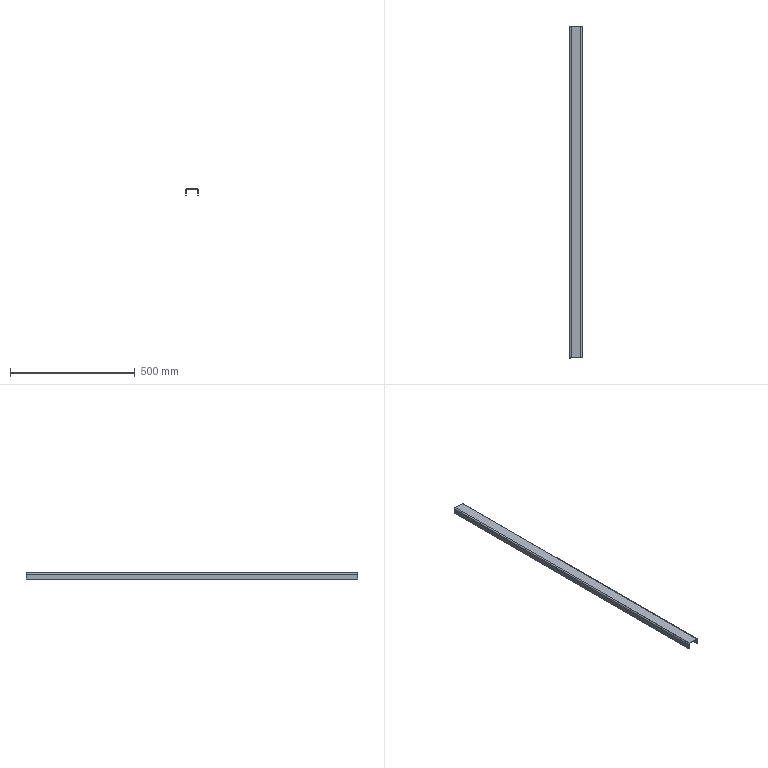Component | SolidWorks | BoxWelding-1_SupportChannelPlate-1 | 1 solid | 14 faces | box 50 x 1331 x 25 mm | volume 246412 mm3 | plane 10 | cylinder 4 | commonest cylinder face diameters 10 x2 6 x2
build123d program:
from build123d import *

# Parameters (mm, degrees)
EXTRUDE_THIN1_DEPTH = 665.5


with BuildPart() as part:
    # Sketch1 → Extrude-Thin1 (new, symmetric)
    with BuildSketch(Plane.XY):
        with BuildLine():
            Line((-25, 24), (-25, 4))
            ThreePointArc((-25, 4), (-23.536, 0.4645), (-20, -1))
            Line((-20, -1), (20, -1))
            ThreePointArc((20, -1), (23.536, 0.4645), (25, 4))
            Line((25, 4), (25, 24))
            Line((25, 24), (23, 24))
            Line((23, 24), (23, 4))
            ThreePointArc((23, 4), (22.121, 1.879), (20, 1))
            Line((20, 1), (-20, 1))
            ThreePointArc((-20, 1), (-22.121, 1.879), (-23, 4))
            Line((-23, 4), (-23, 24))
            Line((-23, 24), (-25, 24))
        make_face()
    extrude(amount=EXTRUDE_THIN1_DEPTH, both=True)


solid = part.part

# Placed as in the assembly
solid = solid.moved(Location((-103.378, 621.001, -155.987), (-90, 0, 0)))
STEP:
#1=COLOUR_RGB('',0.7922,0.8196,0.9333);
#2=FILL_AREA_STYLE_COLOUR('',#1);
#3=FILL_AREA_STYLE('',(#2));
#4=SURFACE_STYLE_FILL_AREA(#3);
#5=SURFACE_SIDE_STYLE('',(#4));
#6=SURFACE_STYLE_USAGE(.BOTH.,#5);
#7=PRESENTATION_STYLE_ASSIGNMENT((#6));
#8=CARTESIAN_POINT('',(-3.165,50.65,-6.299));
#9=VERTEX_POINT('',#8);
#10=CARTESIAN_POINT('',(-3.165,50.65,-7.086));
#11=VERTEX_POINT('',#10);
#12=CARTESIAN_POINT('',(-3.165,50.65,-7.086));
#13=DIRECTION('',(0.,-0.,-1.));
#14=VECTOR('',#13,39.37);
#15=LINE('',#12,#14);
#16=EDGE_CURVE('',#9,#11,#15,.T.);
#17=ORIENTED_EDGE('',*,*,#16,.T.);
#18=CARTESIAN_POINT('',(-3.165,-1.752,-7.086));
#19=VERTEX_POINT('',#18);
#20=CARTESIAN_POINT('',(-3.165,-1.752,-7.086));
#21=DIRECTION('',(-0.,1.,-0.));
#22=VECTOR('',#21,39.37);
#23=LINE('',#20,#22);
#24=EDGE_CURVE('',#19,#11,#23,.T.);
#25=ORIENTED_EDGE('',*,*,#24,.F.);
#26=CARTESIAN_POINT('',(-3.165,-1.752,-6.299));
#27=VERTEX_POINT('',#26);
#28=CARTESIAN_POINT('',(-3.165,-1.752,-7.086));
#29=DIRECTION('',(0.,-0.,-1.));
#30=VECTOR('',#29,39.37);
#31=LINE('',#28,#30);
#32=EDGE_CURVE('',#27,#19,#31,.T.);
#33=ORIENTED_EDGE('',*,*,#32,.F.);
#34=CARTESIAN_POINT('',(-3.165,-1.752,-6.299));
#35=DIRECTION('',(-0.,1.,-0.));
#36=VECTOR('',#35,39.37);
#37=LINE('',#34,#36);
#38=EDGE_CURVE('',#27,#9,#37,.T.);
#39=ORIENTED_EDGE('',*,*,#38,.T.);
#40=EDGE_LOOP('',(#17,#25,#33,#39));
#41=FACE_OUTER_BOUND('',#40,.T.);
#42=CARTESIAN_POINT('',(-3.165,-1.752,-7.086));
#43=DIRECTION('',(1.,0.,0.));
#44=DIRECTION('',(0.,-1.,0.));
#45=AXIS2_PLACEMENT_3D('',#42,#43,#44);
#46=PLANE('',#45);
#47=ADVANCED_FACE('',(#41),#46,.F.);
#48=CARTESIAN_POINT('',(-3.086,50.65,-7.086));
#49=VERTEX_POINT('',#48);
#50=CARTESIAN_POINT('',(-3.086,50.65,-7.086));
#51=DIRECTION('',(-1.,-0.,-0.));
#52=VECTOR('',#51,39.37);
#53=LINE('',#50,#52);
#54=EDGE_CURVE('',#49,#11,#53,.T.);
#55=ORIENTED_EDGE('',*,*,#54,.F.);
#56=CARTESIAN_POINT('',(-3.086,-1.752,-7.086));
#57=VERTEX_POINT('',#56);
#58=CARTESIAN_POINT('',(-3.086,-1.752,-7.086));
#59=DIRECTION('',(-0.,1.,-0.));
#60=VECTOR('',#59,39.37);
#61=LINE('',#58,#60);
#62=EDGE_CURVE('',#57,#49,#61,.T.);
#63=ORIENTED_EDGE('',*,*,#62,.F.);
#64=CARTESIAN_POINT('',(-3.086,-1.752,-7.086));
#65=DIRECTION('',(-1.,-0.,-0.));
#66=VECTOR('',#65,39.37);
#67=LINE('',#64,#66);
#68=EDGE_CURVE('',#57,#19,#67,.T.);
#69=ORIENTED_EDGE('',*,*,#68,.T.);
#70=ORIENTED_EDGE('',*,*,#24,.T.);
#71=EDGE_LOOP('',(#55,#63,#69,#70));
#72=FACE_OUTER_BOUND('',#71,.T.);
#73=CARTESIAN_POINT('',(-3.086,-1.752,-7.086));
#74=DIRECTION('',(0.,-0.,-1.));
#75=DIRECTION('',(0.,-1.,0.));
#76=AXIS2_PLACEMENT_3D('',#73,#74,#75);
#77=PLANE('',#76);
#78=ADVANCED_FACE('',(#72),#77,.T.);
#79=CARTESIAN_POINT('',(-3.086,50.65,-6.299));
#80=VERTEX_POINT('',#79);
#81=CARTESIAN_POINT('',(-3.086,50.65,-7.086));
#82=DIRECTION('',(0.,-0.,-1.));
#83=VECTOR('',#82,39.37);
#84=LINE('',#81,#83);
#85=EDGE_CURVE('',#80,#49,#84,.T.);
#86=ORIENTED_EDGE('',*,*,#85,.F.);
#87=CARTESIAN_POINT('',(-3.086,-1.752,-6.299));
#88=VERTEX_POINT('',#87);
#89=CARTESIAN_POINT('',(-3.086,-1.752,-6.299));
#90=DIRECTION('',(-0.,1.,-0.));
#91=VECTOR('',#90,39.37);
#92=LINE('',#89,#91);
#93=EDGE_CURVE('',#88,#80,#92,.T.);
#94=ORIENTED_EDGE('',*,*,#93,.F.);
#95=CARTESIAN_POINT('',(-3.086,-1.752,-7.086));
#96=DIRECTION('',(0.,-0.,-1.));
#97=VECTOR('',#96,39.37);
#98=LINE('',#95,#97);
#99=EDGE_CURVE('',#88,#57,#98,.T.);
#100=ORIENTED_EDGE('',*,*,#99,.T.);
#101=ORIENTED_EDGE('',*,*,#62,.T.);
#102=EDGE_LOOP('',(#86,#94,#100,#101));
#103=FACE_OUTER_BOUND('',#102,.T.);
#104=CARTESIAN_POINT('',(-3.086,-1.752,-7.086));
#105=DIRECTION('',(1.,0.,0.));
#106=DIRECTION('',(0.,-1.,0.));
#107=AXIS2_PLACEMENT_3D('',#104,#105,#106);
#108=PLANE('',#107);
#109=ADVANCED_FACE('',(#103),#108,.T.);
#110=CARTESIAN_POINT('',(-3.283,50.65,-6.102));
#111=VERTEX_POINT('',#110);
#112=CARTESIAN_POINT('',(-3.283,50.65,-6.299));
#113=DIRECTION('',(-0.,1.,-0.));
#114=DIRECTION('',(-1.,0.,-0.));
#115=AXIS2_PLACEMENT_3D('',#112,#113,#114);
#116=CIRCLE('',#115,0.1969);
#117=EDGE_CURVE('',#111,#80,#116,.T.);
#118=ORIENTED_EDGE('',*,*,#117,.F.);
#119=CARTESIAN_POINT('',(-3.283,-1.752,-6.102));
#120=VERTEX_POINT('',#119);
#121=CARTESIAN_POINT('',(-3.283,-1.752,-6.102));
#122=DIRECTION('',(-0.,1.,-0.));
#123=VECTOR('',#122,39.37);
#124=LINE('',#121,#123);
#125=EDGE_CURVE('',#120,#111,#124,.T.);
#126=ORIENTED_EDGE('',*,*,#125,.F.);
#127=CARTESIAN_POINT('',(-3.283,-1.752,-6.299));
#128=DIRECTION('',(-0.,1.,-0.));
#129=DIRECTION('',(-1.,-0.,-0.));
#130=AXIS2_PLACEMENT_3D('',#127,#128,#129);
#131=CIRCLE('',#130,0.1969);
#132=EDGE_CURVE('',#120,#88,#131,.T.);
#133=ORIENTED_EDGE('',*,*,#132,.T.);
#134=ORIENTED_EDGE('',*,*,#93,.T.);
#135=EDGE_LOOP('',(#118,#126,#133,#134));
#136=FACE_OUTER_BOUND('',#135,.T.);
#137=CARTESIAN_POINT('',(-3.283,-1.752,-6.299));
#138=DIRECTION('',(-0.,1.,-0.));
#139=DIRECTION('',(1.,0.,0.));
#140=AXIS2_PLACEMENT_3D('',#137,#138,#139);
#141=CYLINDRICAL_SURFACE('',#140,0.1969);
#142=ADVANCED_FACE('',(#136),#141,.T.);
#143=CARTESIAN_POINT('',(-4.857,50.65,-6.102));
#144=VERTEX_POINT('',#143);
#145=CARTESIAN_POINT('',(-3.283,50.65,-6.102));
#146=DIRECTION('',(1.,0.,0.));
#147=VECTOR('',#146,39.37);
#148=LINE('',#145,#147);
#149=EDGE_CURVE('',#144,#111,#148,.T.);
#150=ORIENTED_EDGE('',*,*,#149,.F.);
#151=CARTESIAN_POINT('',(-4.857,-1.752,-6.102));
#152=VERTEX_POINT('',#151);
#153=CARTESIAN_POINT('',(-4.857,-1.752,-6.102));
#154=DIRECTION('',(-0.,1.,-0.));
#155=VECTOR('',#154,39.37);
#156=LINE('',#153,#155);
#157=EDGE_CURVE('',#152,#144,#156,.T.);
#158=ORIENTED_EDGE('',*,*,#157,.F.);
#159=CARTESIAN_POINT('',(-3.283,-1.752,-6.102));
#160=DIRECTION('',(1.,0.,0.));
#161=VECTOR('',#160,39.37);
#162=LINE('',#159,#161);
#163=EDGE_CURVE('',#152,#120,#162,.T.);
#164=ORIENTED_EDGE('',*,*,#163,.T.);
#165=ORIENTED_EDGE('',*,*,#125,.T.);
#166=EDGE_LOOP('',(#150,#158,#164,#165));
#167=FACE_OUTER_BOUND('',#166,.T.);
#168=CARTESIAN_POINT('',(-3.283,-1.752,-6.102));
#169=DIRECTION('',(-0.,0.,1.));
#170=DIRECTION('',(-0.,1.,-0.));
#171=AXIS2_PLACEMENT_3D('',#168,#169,#170);
#172=PLANE('',#171);
#173=ADVANCED_FACE('',(#167),#172,.T.);
#174=CARTESIAN_POINT('',(-5.054,50.65,-6.299));
#175=VERTEX_POINT('',#174);
#176=CARTESIAN_POINT('',(-4.857,50.65,-6.299));
#177=DIRECTION('',(-0.,1.,-0.));
#178=DIRECTION('',(-1.,0.,0.));
#179=AXIS2_PLACEMENT_3D('',#176,#177,#178);
#180=CIRCLE('',#179,0.1969);
#181=EDGE_CURVE('',#175,#144,#180,.T.);
#182=ORIENTED_EDGE('',*,*,#181,.F.);
#183=CARTESIAN_POINT('',(-5.054,-1.752,-6.299));
#184=VERTEX_POINT('',#183);
#185=CARTESIAN_POINT('',(-5.054,-1.752,-6.299));
#186=DIRECTION('',(-0.,1.,-0.));
#187=VECTOR('',#186,39.37);
#188=LINE('',#185,#187);
#189=EDGE_CURVE('',#184,#175,#188,.T.);
#190=ORIENTED_EDGE('',*,*,#189,.F.);
#191=CARTESIAN_POINT('',(-4.857,-1.752,-6.299));
#192=DIRECTION('',(-0.,1.,-0.));
#193=DIRECTION('',(-1.,-0.,0.));
#194=AXIS2_PLACEMENT_3D('',#191,#192,#193);
#195=CIRCLE('',#194,0.1969);
#196=EDGE_CURVE('',#184,#152,#195,.T.);
#197=ORIENTED_EDGE('',*,*,#196,.T.);
#198=ORIENTED_EDGE('',*,*,#157,.T.);
#199=EDGE_LOOP('',(#182,#190,#197,#198));
#200=FACE_OUTER_BOUND('',#199,.T.);
#201=CARTESIAN_POINT('',(-4.857,-1.752,-6.299));
#202=DIRECTION('',(-0.,1.,-0.));
#203=DIRECTION('',(1.,0.,0.));
#204=AXIS2_PLACEMENT_3D('',#201,#202,#203);
#205=CYLINDRICAL_SURFACE('',#204,0.1969);
#206=ADVANCED_FACE('',(#200),#205,.T.);
#207=CARTESIAN_POINT('',(-5.054,50.65,-7.086));
#208=VERTEX_POINT('',#207);
#209=CARTESIAN_POINT('',(-5.054,50.65,-7.086));
#210=DIRECTION('',(-0.,0.,1.));
#211=VECTOR('',#210,39.37);
#212=LINE('',#209,#211);
#213=EDGE_CURVE('',#208,#175,#212,.T.);
#214=ORIENTED_EDGE('',*,*,#213,.F.);
#215=CARTESIAN_POINT('',(-5.054,-1.752,-7.086));
#216=VERTEX_POINT('',#215);
#217=CARTESIAN_POINT('',(-5.054,-1.752,-7.086));
#218=DIRECTION('',(-0.,1.,-0.));
#219=VECTOR('',#218,39.37);
#220=LINE('',#217,#219);
#221=EDGE_CURVE('',#216,#208,#220,.T.);
#222=ORIENTED_EDGE('',*,*,#221,.F.);
#223=CARTESIAN_POINT('',(-5.054,-1.752,-7.086));
#224=DIRECTION('',(-0.,0.,1.));
#225=VECTOR('',#224,39.37);
#226=LINE('',#223,#225);
#227=EDGE_CURVE('',#216,#184,#226,.T.);
#228=ORIENTED_EDGE('',*,*,#227,.T.);
#229=ORIENTED_EDGE('',*,*,#189,.T.);
#230=EDGE_LOOP('',(#214,#222,#228,#229));
#231=FACE_OUTER_BOUND('',#230,.T.);
#232=CARTESIAN_POINT('',(-5.054,-1.752,-7.086));
#233=DIRECTION('',(-1.,-0.,-0.));
#234=DIRECTION('',(-0.,1.,-0.));
#235=AXIS2_PLACEMENT_3D('',#232,#233,#234);
#236=PLANE('',#235);
#237=ADVANCED_FACE('',(#231),#236,.T.);
#238=CARTESIAN_POINT('',(-4.976,50.65,-7.086));
#239=VERTEX_POINT('',#238);
#240=CARTESIAN_POINT('',(-4.976,50.65,-7.086));
#241=DIRECTION('',(-1.,-0.,-0.));
#242=VECTOR('',#241,39.37);
#243=LINE('',#240,#242);
#244=EDGE_CURVE('',#239,#208,#243,.T.);
#245=ORIENTED_EDGE('',*,*,#244,.F.);
#246=CARTESIAN_POINT('',(-4.976,-1.752,-7.086));
#247=VERTEX_POINT('',#246);
#248=CARTESIAN_POINT('',(-4.976,-1.752,-7.086));
#249=DIRECTION('',(-0.,1.,-0.));
#250=VECTOR('',#249,39.37);
#251=LINE('',#248,#250);
#252=EDGE_CURVE('',#247,#239,#251,.T.);
#253=ORIENTED_EDGE('',*,*,#252,.F.);
#254=CARTESIAN_POINT('',(-4.976,-1.752,-7.086));
#255=DIRECTION('',(-1.,-0.,-0.));
#256=VECTOR('',#255,39.37);
#257=LINE('',#254,#256);
#258=EDGE_CURVE('',#247,#216,#257,.T.);
#259=ORIENTED_EDGE('',*,*,#258,.T.);
#260=ORIENTED_EDGE('',*,*,#221,.T.);
#261=EDGE_LOOP('',(#245,#253,#259,#260));
#262=FACE_OUTER_BOUND('',#261,.T.);
#263=CARTESIAN_POINT('',(-4.976,-1.752,-7.086));
#264=DIRECTION('',(0.,-0.,-1.));
#265=DIRECTION('',(0.,-1.,0.));
#266=AXIS2_PLACEMENT_3D('',#263,#264,#265);
#267=PLANE('',#266);
#268=ADVANCED_FACE('',(#262),#267,.T.);
#269=CARTESIAN_POINT('',(-4.976,50.65,-6.299));
#270=VERTEX_POINT('',#269);
#271=CARTESIAN_POINT('',(-4.976,50.65,-7.086));
#272=DIRECTION('',(-0.,0.,1.));
#273=VECTOR('',#272,39.37);
#274=LINE('',#271,#273);
#275=EDGE_CURVE('',#239,#270,#274,.T.);
#276=ORIENTED_EDGE('',*,*,#275,.T.);
#277=CARTESIAN_POINT('',(-4.976,-1.752,-6.299));
#278=VERTEX_POINT('',#277);
#279=CARTESIAN_POINT('',(-4.976,-1.752,-6.299));
#280=DIRECTION('',(-0.,1.,-0.));
#281=VECTOR('',#280,39.37);
#282=LINE('',#279,#281);
#283=EDGE_CURVE('',#278,#270,#282,.T.);
#284=ORIENTED_EDGE('',*,*,#283,.F.);
#285=CARTESIAN_POINT('',(-4.976,-1.752,-7.086));
#286=DIRECTION('',(-0.,0.,1.));
#287=VECTOR('',#286,39.37);
#288=LINE('',#285,#287);
#289=EDGE_CURVE('',#247,#278,#288,.T.);
#290=ORIENTED_EDGE('',*,*,#289,.F.);
#291=ORIENTED_EDGE('',*,*,#252,.T.);
#292=EDGE_LOOP('',(#276,#284,#290,#291));
#293=FACE_OUTER_BOUND('',#292,.T.);
#294=CARTESIAN_POINT('',(-4.976,-1.752,-7.086));
#295=DIRECTION('',(-1.,-0.,-0.));
#296=DIRECTION('',(-0.,1.,-0.));
#297=AXIS2_PLACEMENT_3D('',#294,#295,#296);
#298=PLANE('',#297);
#299=ADVANCED_FACE('',(#293),#298,.F.);
#300=CARTESIAN_POINT('',(-4.857,50.65,-6.181));
#301=VERTEX_POINT('',#300);
#302=CARTESIAN_POINT('',(-4.857,50.65,-6.299));
#303=DIRECTION('',(-0.,1.,-0.));
#304=DIRECTION('',(-1.,0.,0.));
#305=AXIS2_PLACEMENT_3D('',#302,#303,#304);
#306=CIRCLE('',#305,0.1181);
#307=EDGE_CURVE('',#270,#301,#306,.T.);
#308=ORIENTED_EDGE('',*,*,#307,.T.);
#309=CARTESIAN_POINT('',(-4.857,-1.752,-6.181));
#310=VERTEX_POINT('',#309);
#311=CARTESIAN_POINT('',(-4.857,-1.752,-6.181));
#312=DIRECTION('',(-0.,1.,-0.));
#313=VECTOR('',#312,39.37);
#314=LINE('',#311,#313);
#315=EDGE_CURVE('',#310,#301,#314,.T.);
#316=ORIENTED_EDGE('',*,*,#315,.F.);
#317=CARTESIAN_POINT('',(-4.857,-1.752,-6.299));
#318=DIRECTION('',(-0.,1.,-0.));
#319=DIRECTION('',(-1.,-0.,0.));
#320=AXIS2_PLACEMENT_3D('',#317,#318,#319);
#321=CIRCLE('',#320,0.1181);
#322=EDGE_CURVE('',#278,#310,#321,.T.);
#323=ORIENTED_EDGE('',*,*,#322,.F.);
#324=ORIENTED_EDGE('',*,*,#283,.T.);
#325=EDGE_LOOP('',(#308,#316,#323,#324));
#326=FACE_OUTER_BOUND('',#325,.T.);
#327=CARTESIAN_POINT('',(-4.857,-1.752,-6.299));
#328=DIRECTION('',(-0.,1.,-0.));
#329=DIRECTION('',(1.,0.,0.));
#330=AXIS2_PLACEMENT_3D('',#327,#328,#329);
#331=CYLINDRICAL_SURFACE('',#330,0.1181);
#332=ADVANCED_FACE('',(#326),#331,.F.);
#333=CARTESIAN_POINT('',(-3.283,50.65,-6.181));
#334=VERTEX_POINT('',#333);
#335=CARTESIAN_POINT('',(-3.283,50.65,-6.181));
#336=DIRECTION('',(1.,0.,0.));
#337=VECTOR('',#336,39.37);
#338=LINE('',#335,#337);
#339=EDGE_CURVE('',#301,#334,#338,.T.);
#340=ORIENTED_EDGE('',*,*,#339,.T.);
#341=CARTESIAN_POINT('',(-3.283,-1.752,-6.181));
#342=VERTEX_POINT('',#341);
#343=CARTESIAN_POINT('',(-3.283,-1.752,-6.181));
#344=DIRECTION('',(-0.,1.,-0.));
#345=VECTOR('',#344,39.37);
#346=LINE('',#343,#345);
#347=EDGE_CURVE('',#342,#334,#346,.T.);
#348=ORIENTED_EDGE('',*,*,#347,.F.);
#349=CARTESIAN_POINT('',(-3.283,-1.752,-6.181));
#350=DIRECTION('',(1.,0.,0.));
#351=VECTOR('',#350,39.37);
#352=LINE('',#349,#351);
#353=EDGE_CURVE('',#310,#342,#352,.T.);
#354=ORIENTED_EDGE('',*,*,#353,.F.);
#355=ORIENTED_EDGE('',*,*,#315,.T.);
#356=EDGE_LOOP('',(#340,#348,#354,#355));
#357=FACE_OUTER_BOUND('',#356,.T.);
#358=CARTESIAN_POINT('',(-3.283,-1.752,-6.181));
#359=DIRECTION('',(-0.,0.,1.));
#360=DIRECTION('',(-0.,1.,-0.));
#361=AXIS2_PLACEMENT_3D('',#358,#359,#360);
#362=PLANE('',#361);
#363=ADVANCED_FACE('',(#357),#362,.F.);
#364=CARTESIAN_POINT('',(-3.283,50.65,-6.299));
#365=DIRECTION('',(-0.,1.,-0.));
#366=DIRECTION('',(-1.,0.,0.));
#367=AXIS2_PLACEMENT_3D('',#364,#365,#366);
#368=CIRCLE('',#367,0.1181);
#369=EDGE_CURVE('',#334,#9,#368,.T.);
#370=ORIENTED_EDGE('',*,*,#369,.T.);
#371=ORIENTED_EDGE('',*,*,#38,.F.);
#372=CARTESIAN_POINT('',(-3.283,-1.752,-6.299));
#373=DIRECTION('',(-0.,1.,-0.));
#374=DIRECTION('',(-1.,-0.,0.));
#375=AXIS2_PLACEMENT_3D('',#372,#373,#374);
#376=CIRCLE('',#375,0.1181);
#377=EDGE_CURVE('',#342,#27,#376,.T.);
#378=ORIENTED_EDGE('',*,*,#377,.F.);
#379=ORIENTED_EDGE('',*,*,#347,.T.);
#380=EDGE_LOOP('',(#370,#371,#378,#379));
#381=FACE_OUTER_BOUND('',#380,.T.);
#382=CARTESIAN_POINT('',(-3.283,-1.752,-6.299));
#383=DIRECTION('',(-0.,1.,-0.));
#384=DIRECTION('',(1.,0.,0.));
#385=AXIS2_PLACEMENT_3D('',#382,#383,#384);
#386=CYLINDRICAL_SURFACE('',#385,0.1181);
#387=ADVANCED_FACE('',(#381),#386,.F.);
#388=ORIENTED_EDGE('',*,*,#32,.T.);
#389=ORIENTED_EDGE('',*,*,#68,.F.);
#390=ORIENTED_EDGE('',*,*,#99,.F.);
#391=ORIENTED_EDGE('',*,*,#132,.F.);
#392=ORIENTED_EDGE('',*,*,#163,.F.);
#393=ORIENTED_EDGE('',*,*,#196,.F.);
#394=ORIENTED_EDGE('',*,*,#227,.F.);
#395=ORIENTED_EDGE('',*,*,#258,.F.);
#396=ORIENTED_EDGE('',*,*,#289,.T.);
#397=ORIENTED_EDGE('',*,*,#322,.T.);
#398=ORIENTED_EDGE('',*,*,#353,.T.);
#399=ORIENTED_EDGE('',*,*,#377,.T.);
#400=EDGE_LOOP('',(#388,#389,#390,#391,#392,#393,#394,#395,#396,#397,#398,#399));
#401=FACE_OUTER_BOUND('',#400,.T.);
#402=CARTESIAN_POINT('',(-3.283,-1.752,-6.299));
#403=DIRECTION('',(0.,-1.,0.));
#404=DIRECTION('',(-1.,-0.,-0.));
#405=AXIS2_PLACEMENT_3D('',#402,#403,#404);
#406=PLANE('',#405);
#407=ADVANCED_FACE('',(#401),#406,.T.);
#408=ORIENTED_EDGE('',*,*,#16,.F.);
#409=ORIENTED_EDGE('',*,*,#369,.F.);
#410=ORIENTED_EDGE('',*,*,#339,.F.);
#411=ORIENTED_EDGE('',*,*,#307,.F.);
#412=ORIENTED_EDGE('',*,*,#275,.F.);
#413=ORIENTED_EDGE('',*,*,#244,.T.);
#414=ORIENTED_EDGE('',*,*,#213,.T.);
#415=ORIENTED_EDGE('',*,*,#181,.T.);
#416=ORIENTED_EDGE('',*,*,#149,.T.);
#417=ORIENTED_EDGE('',*,*,#117,.T.);
#418=ORIENTED_EDGE('',*,*,#85,.T.);
#419=ORIENTED_EDGE('',*,*,#54,.T.);
#420=EDGE_LOOP('',(#408,#409,#410,#411,#412,#413,#414,#415,#416,#417,#418,#419));
#421=FACE_OUTER_BOUND('',#420,.T.);
#422=CARTESIAN_POINT('',(-3.283,50.65,-6.299));
#423=DIRECTION('',(0.,-1.,0.));
#424=DIRECTION('',(-1.,-0.,-0.));
#425=AXIS2_PLACEMENT_3D('',#422,#423,#424);
#426=PLANE('',#425);
#427=ADVANCED_FACE('',(#421),#426,.F.);
#428=CLOSED_SHELL('',(#47,#78,#109,#142,#173,#206,#237,#268,#299,#332,#363,#387,#407,#427));
#429=MANIFOLD_SOLID_BREP('',#428);
#430=STYLED_ITEM('',(#7),#429);
#431=PRESENTATION_LAYER_ASSIGNMENT('','',(#430));
#432=CARTESIAN_POINT('',(0.,0.,0.));
#433=DIRECTION('',(0.,0.,1.));
#434=DIRECTION('',(1.,0.,0.));
#435=AXIS2_PLACEMENT_3D('',#432,#433,#434);
#436=(LENGTH_UNIT()NAMED_UNIT(*)SI_UNIT($,.METRE.));
#437=LENGTH_MEASURE_WITH_UNIT(LENGTH_MEASURE(0.0254),#436);
#438=DIMENSIONAL_EXPONENTS(1.,0.,0.,0.,0.,0.,0.);
#439=(CONVERSION_BASED_UNIT('',#437)LENGTH_UNIT()NAMED_UNIT(#438));
#440=UNCERTAINTY_MEASURE_WITH_UNIT(LENGTH_MEASURE(0.00001),#439,'','');
#441=(NAMED_UNIT(*)PLANE_ANGLE_UNIT()SI_UNIT($,.RADIAN.));
#442=(NAMED_UNIT(*)SI_UNIT($,.STERADIAN.)SOLID_ANGLE_UNIT());
#443=(GEOMETRIC_REPRESENTATION_CONTEXT(3)GLOBAL_UNCERTAINTY_ASSIGNED_CONTEXT((#440))GLOBAL_UNIT_ASSIGNED_CONTEXT((#439,#441,#442))REPRESENTATION_CONTEXT('',''));
#444=ADVANCED_BREP_SHAPE_REPRESENTATION('',(#429,#435),#443);
#445=(LENGTH_UNIT()NAMED_UNIT(*)SI_UNIT($,.METRE.));
#446=LENGTH_MEASURE_WITH_UNIT(LENGTH_MEASURE(0.0254),#445);
#447=DIMENSIONAL_EXPONENTS(1.,0.,0.,0.,0.,0.,0.);
#448=(CONVERSION_BASED_UNIT('',#446)LENGTH_UNIT()NAMED_UNIT(#447));
#449=UNCERTAINTY_MEASURE_WITH_UNIT(LENGTH_MEASURE(0.00001),#448,'','');
#450=(NAMED_UNIT(*)PLANE_ANGLE_UNIT()SI_UNIT($,.RADIAN.));
#451=(NAMED_UNIT(*)SI_UNIT($,.STERADIAN.)SOLID_ANGLE_UNIT());
#452=(GEOMETRIC_REPRESENTATION_CONTEXT(3)GLOBAL_UNCERTAINTY_ASSIGNED_CONTEXT((#449))GLOBAL_UNIT_ASSIGNED_CONTEXT((#448,#450,#451))REPRESENTATION_CONTEXT('',''));
#453=MECHANICAL_DESIGN_GEOMETRIC_PRESENTATION_REPRESENTATION('',(#430),#452);